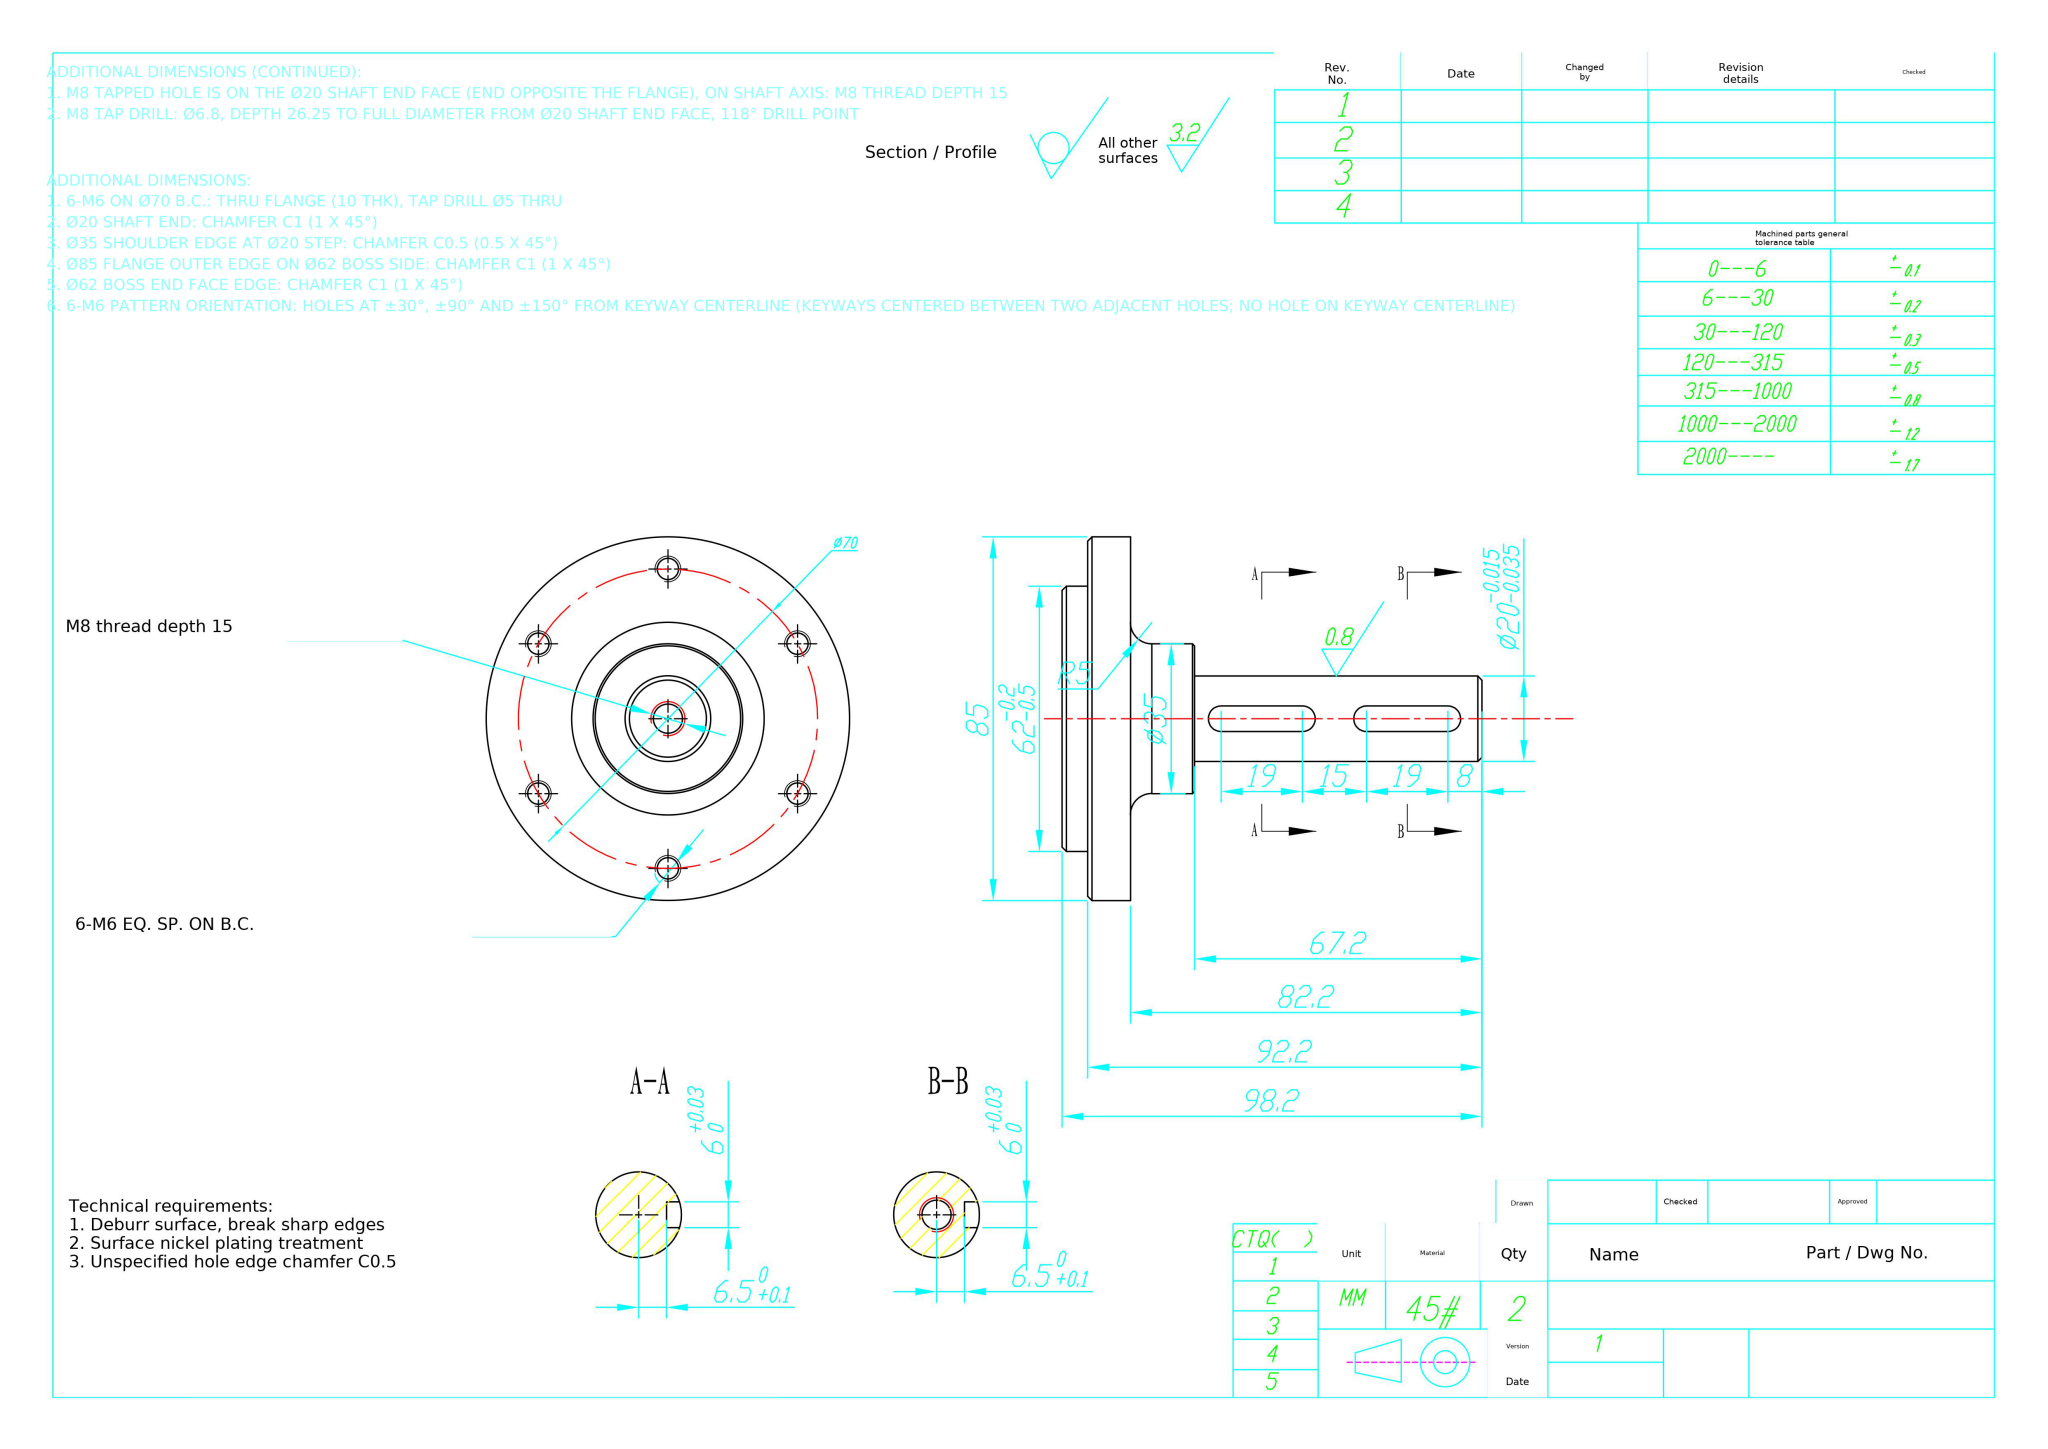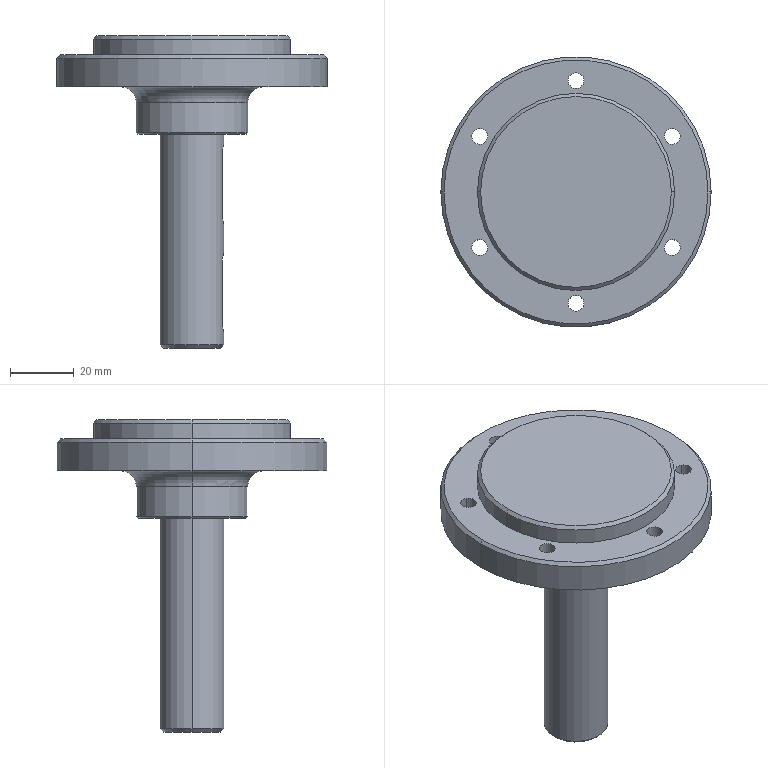Part | NX | mm | 1 solid | 51 faces | box 85 x 85 x 98.2 mm | volume 107646 mm3 | cylinder 28 | plane 11 | cone 10 | torus 2 | commonest cylinder face diameters 5 x12 6 x6 6.8 x2 62 x2 85 x2 35 x2 20 x2